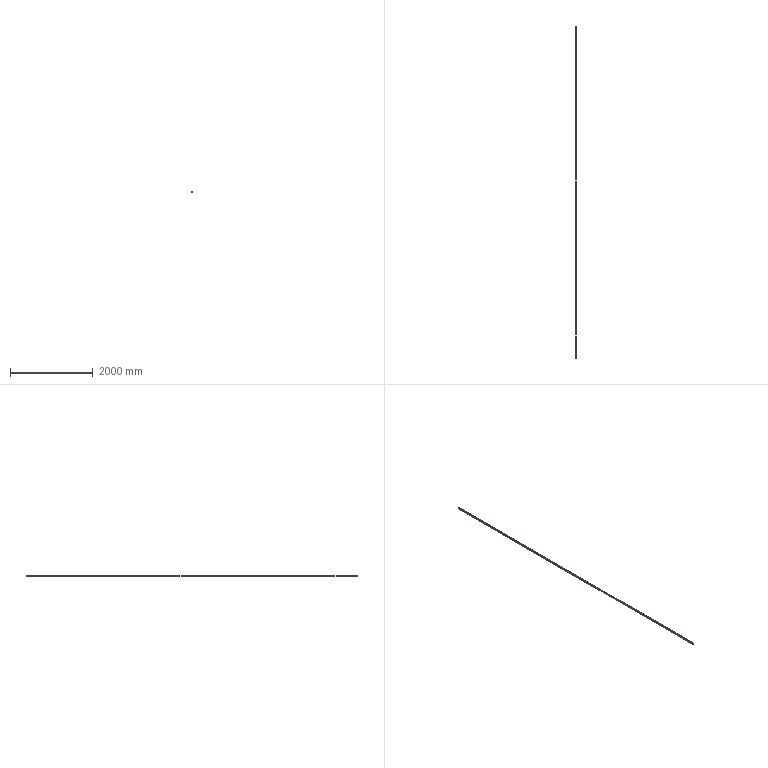Component | SolidWorks | MirrorRailing-10_Mirror30X30X3-7440-2 | 3 solids | 54 faces | volume 2388535 mm3 | plane 30 | cylinder 24 | commonest cylinder face diameters 6 x12 12 x12